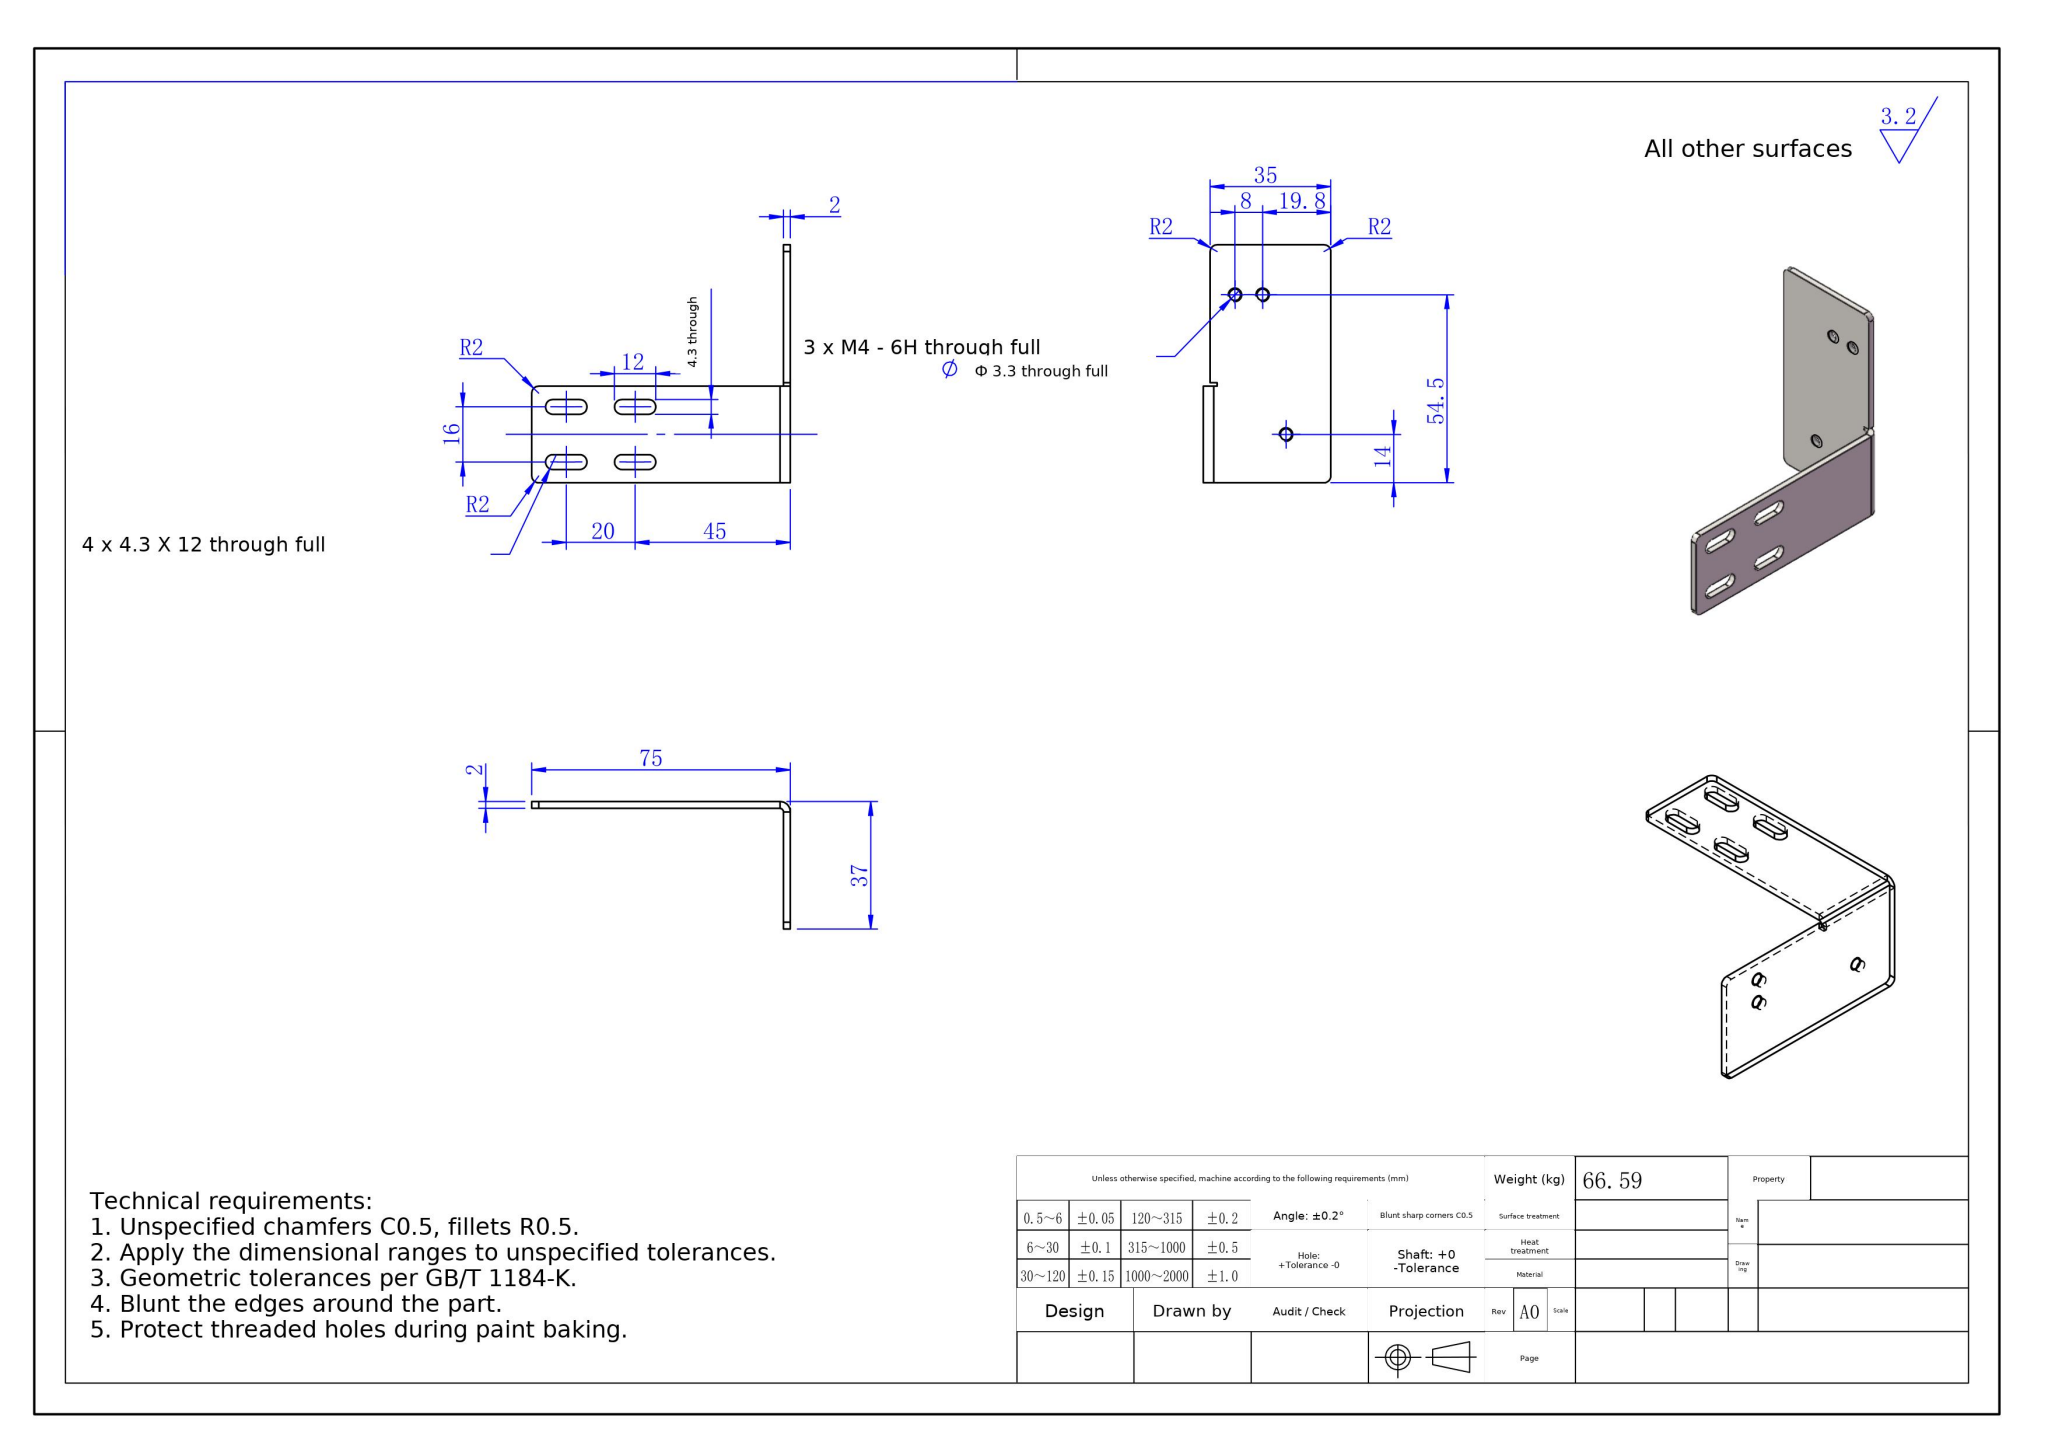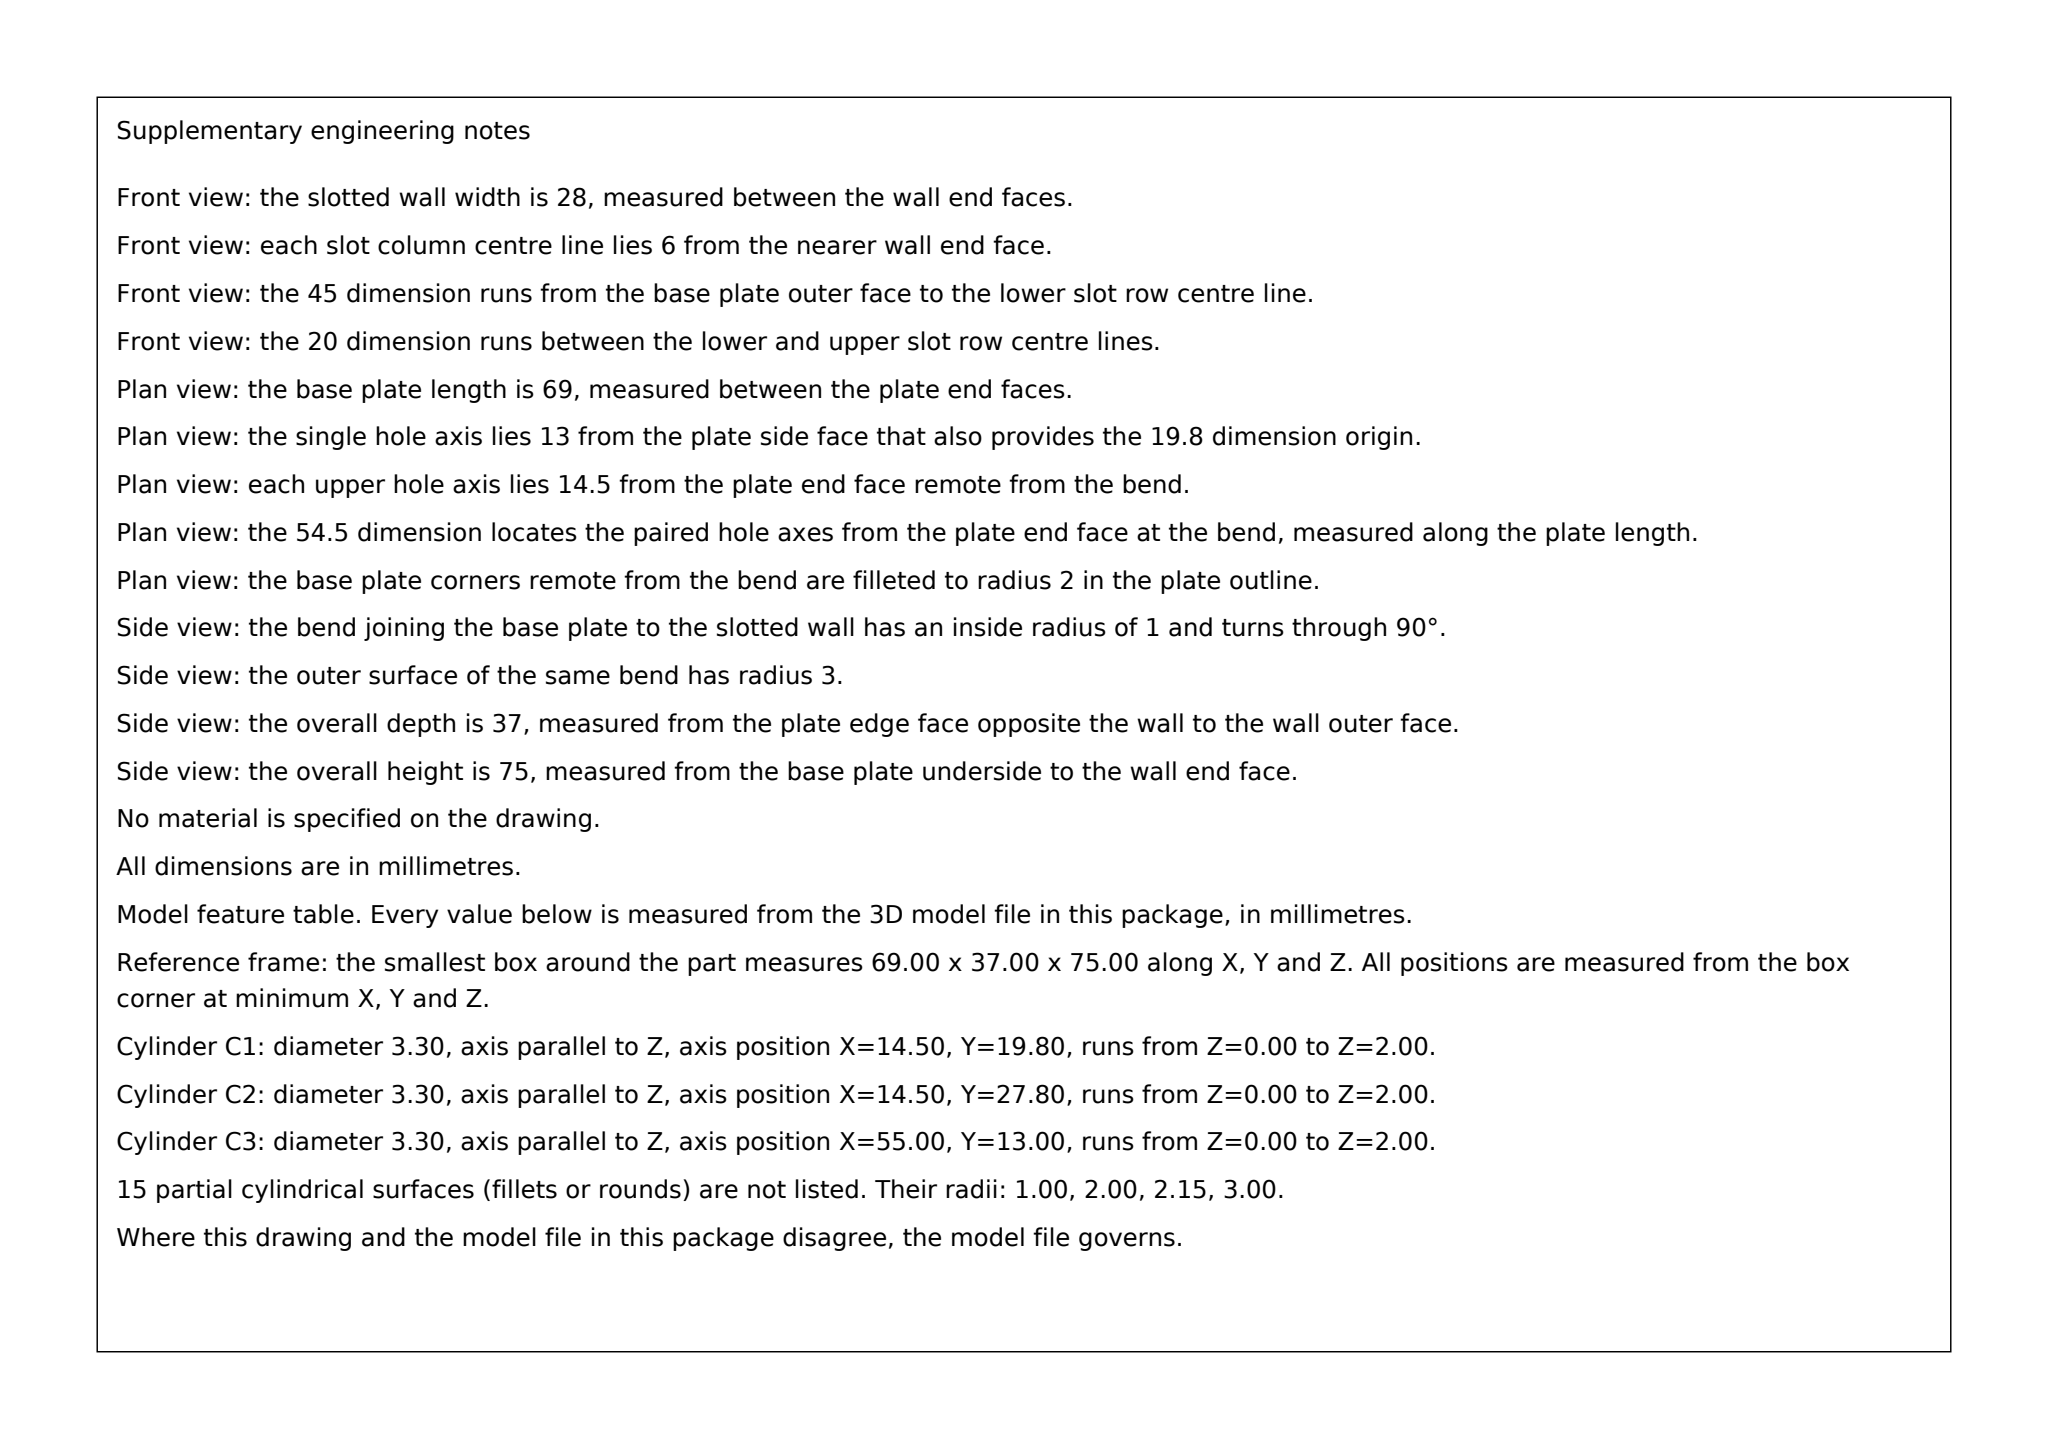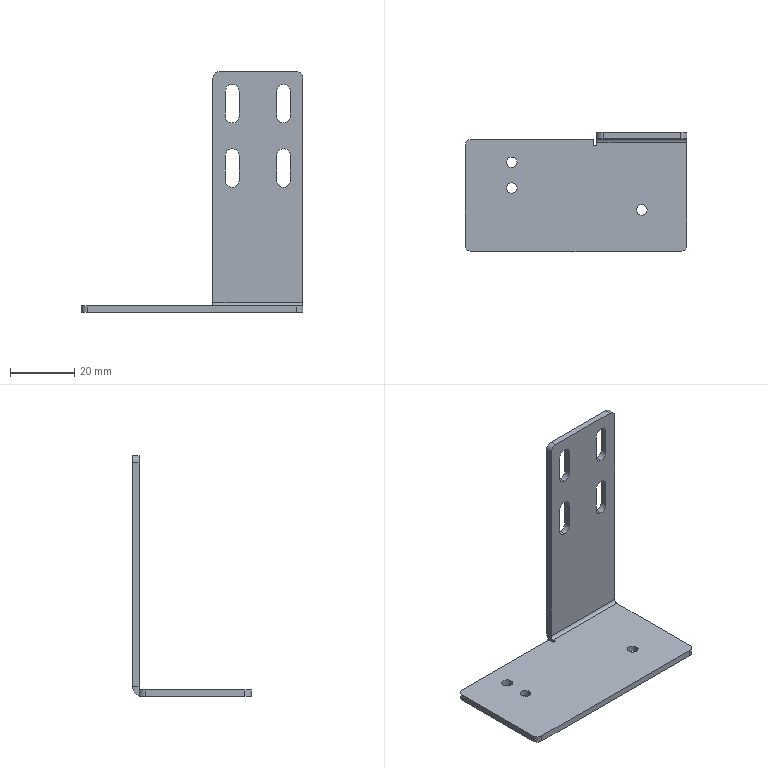Part | SolidWorks | mm | 1 solid | 49 faces | box 69 x 37 x 75 mm | volume 8537 mm3 | cylinder 25 | plane 24 | commonest cylinder face diameters 4.3 x12 3.3 x6 4 x5 6 x1 2 x1